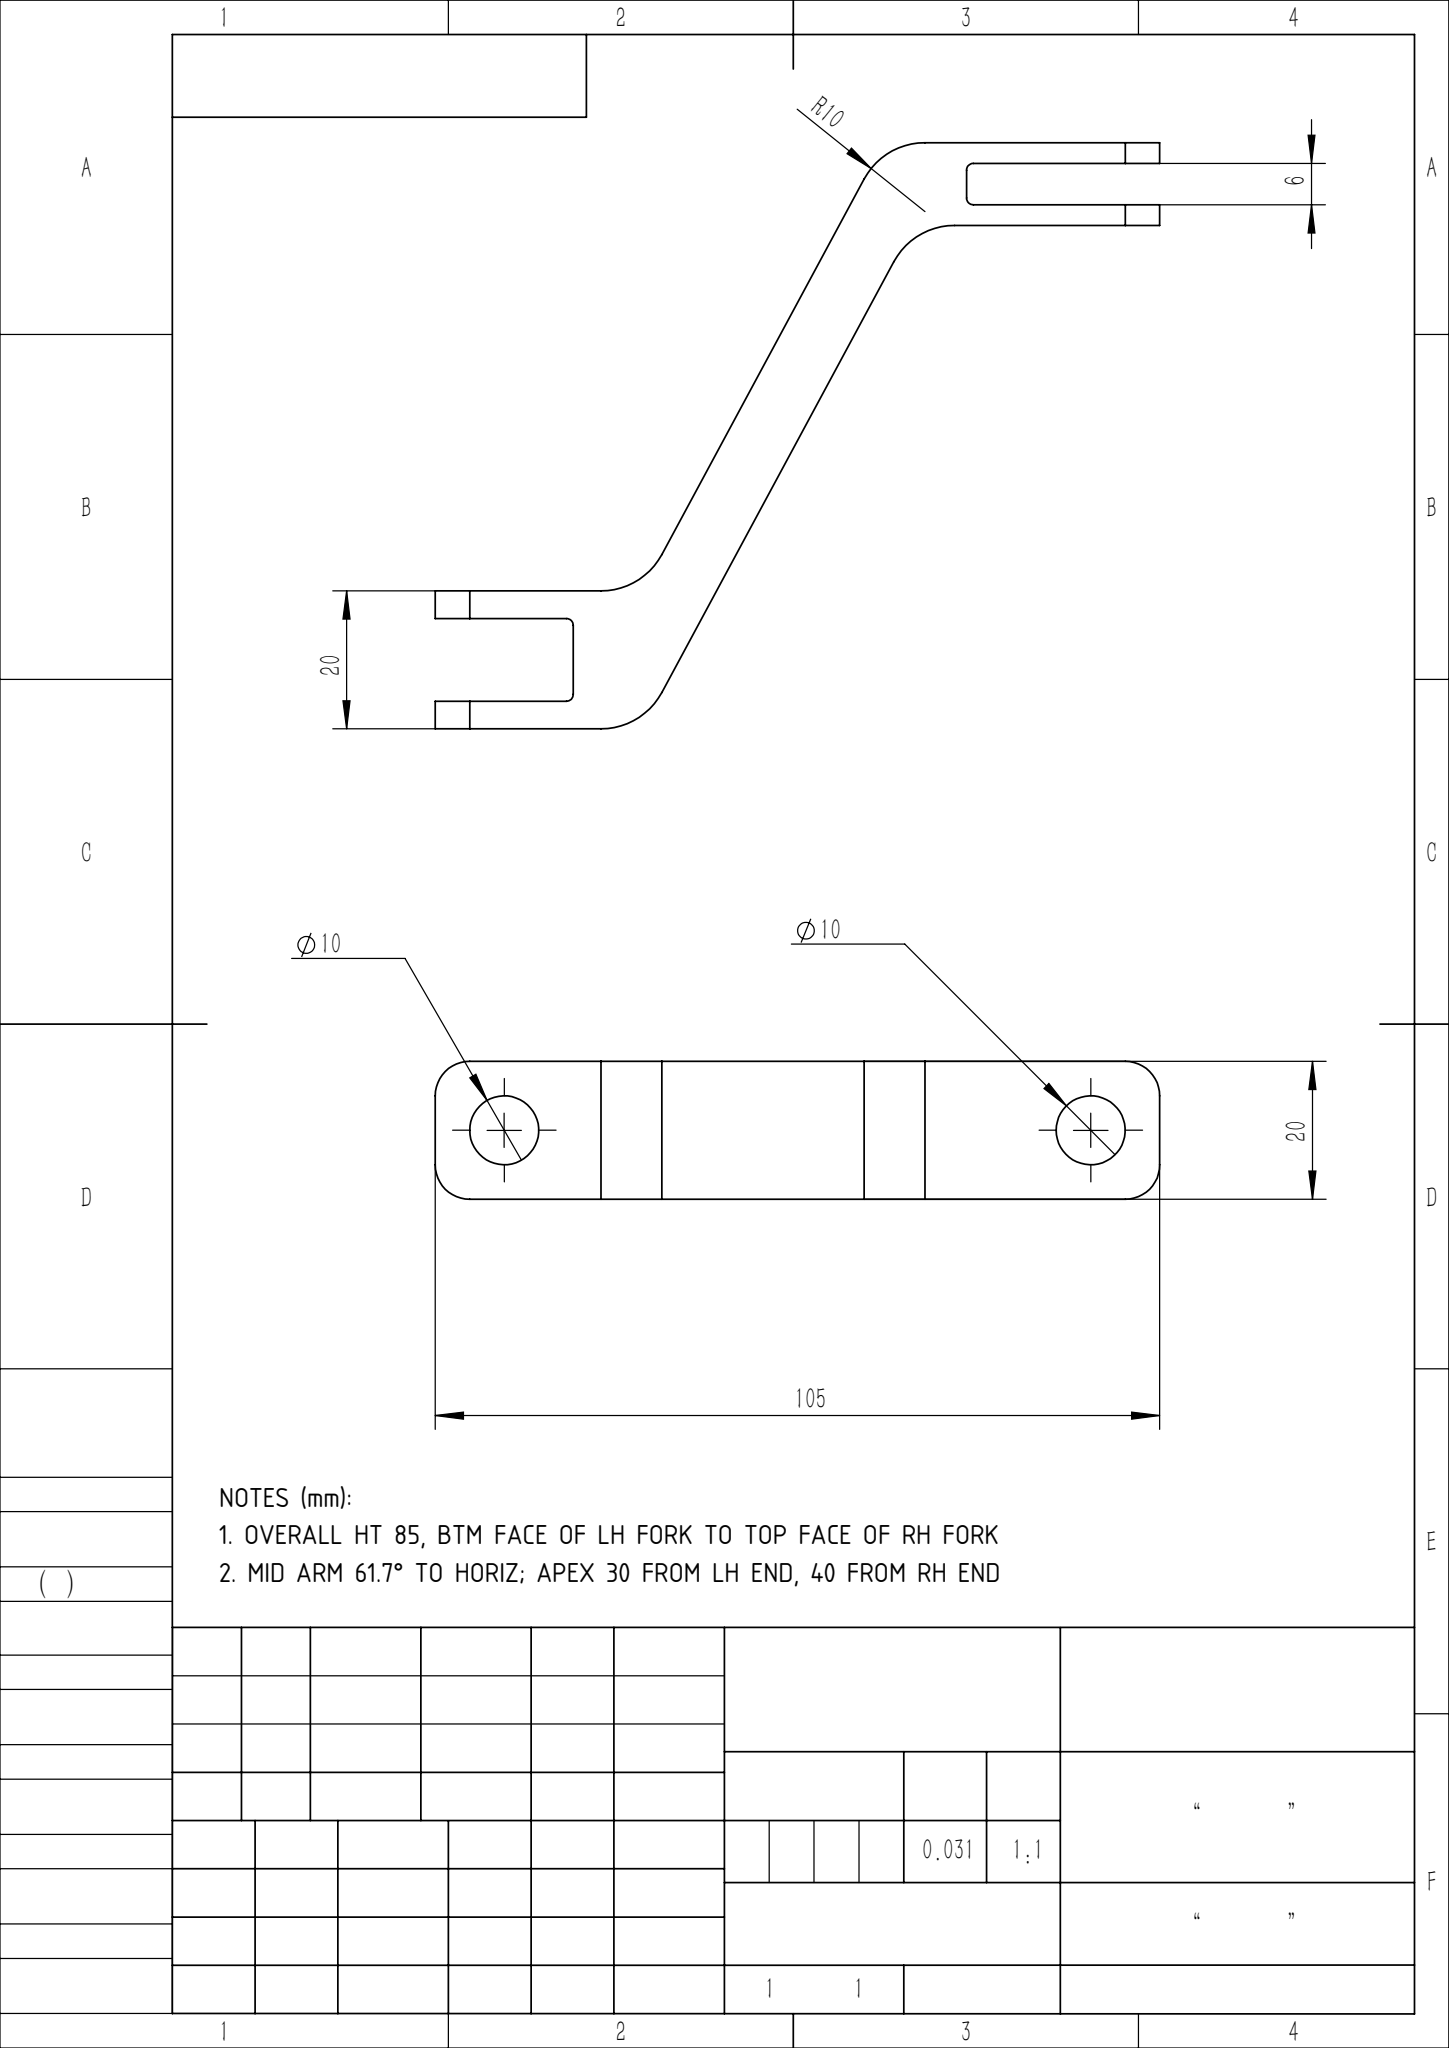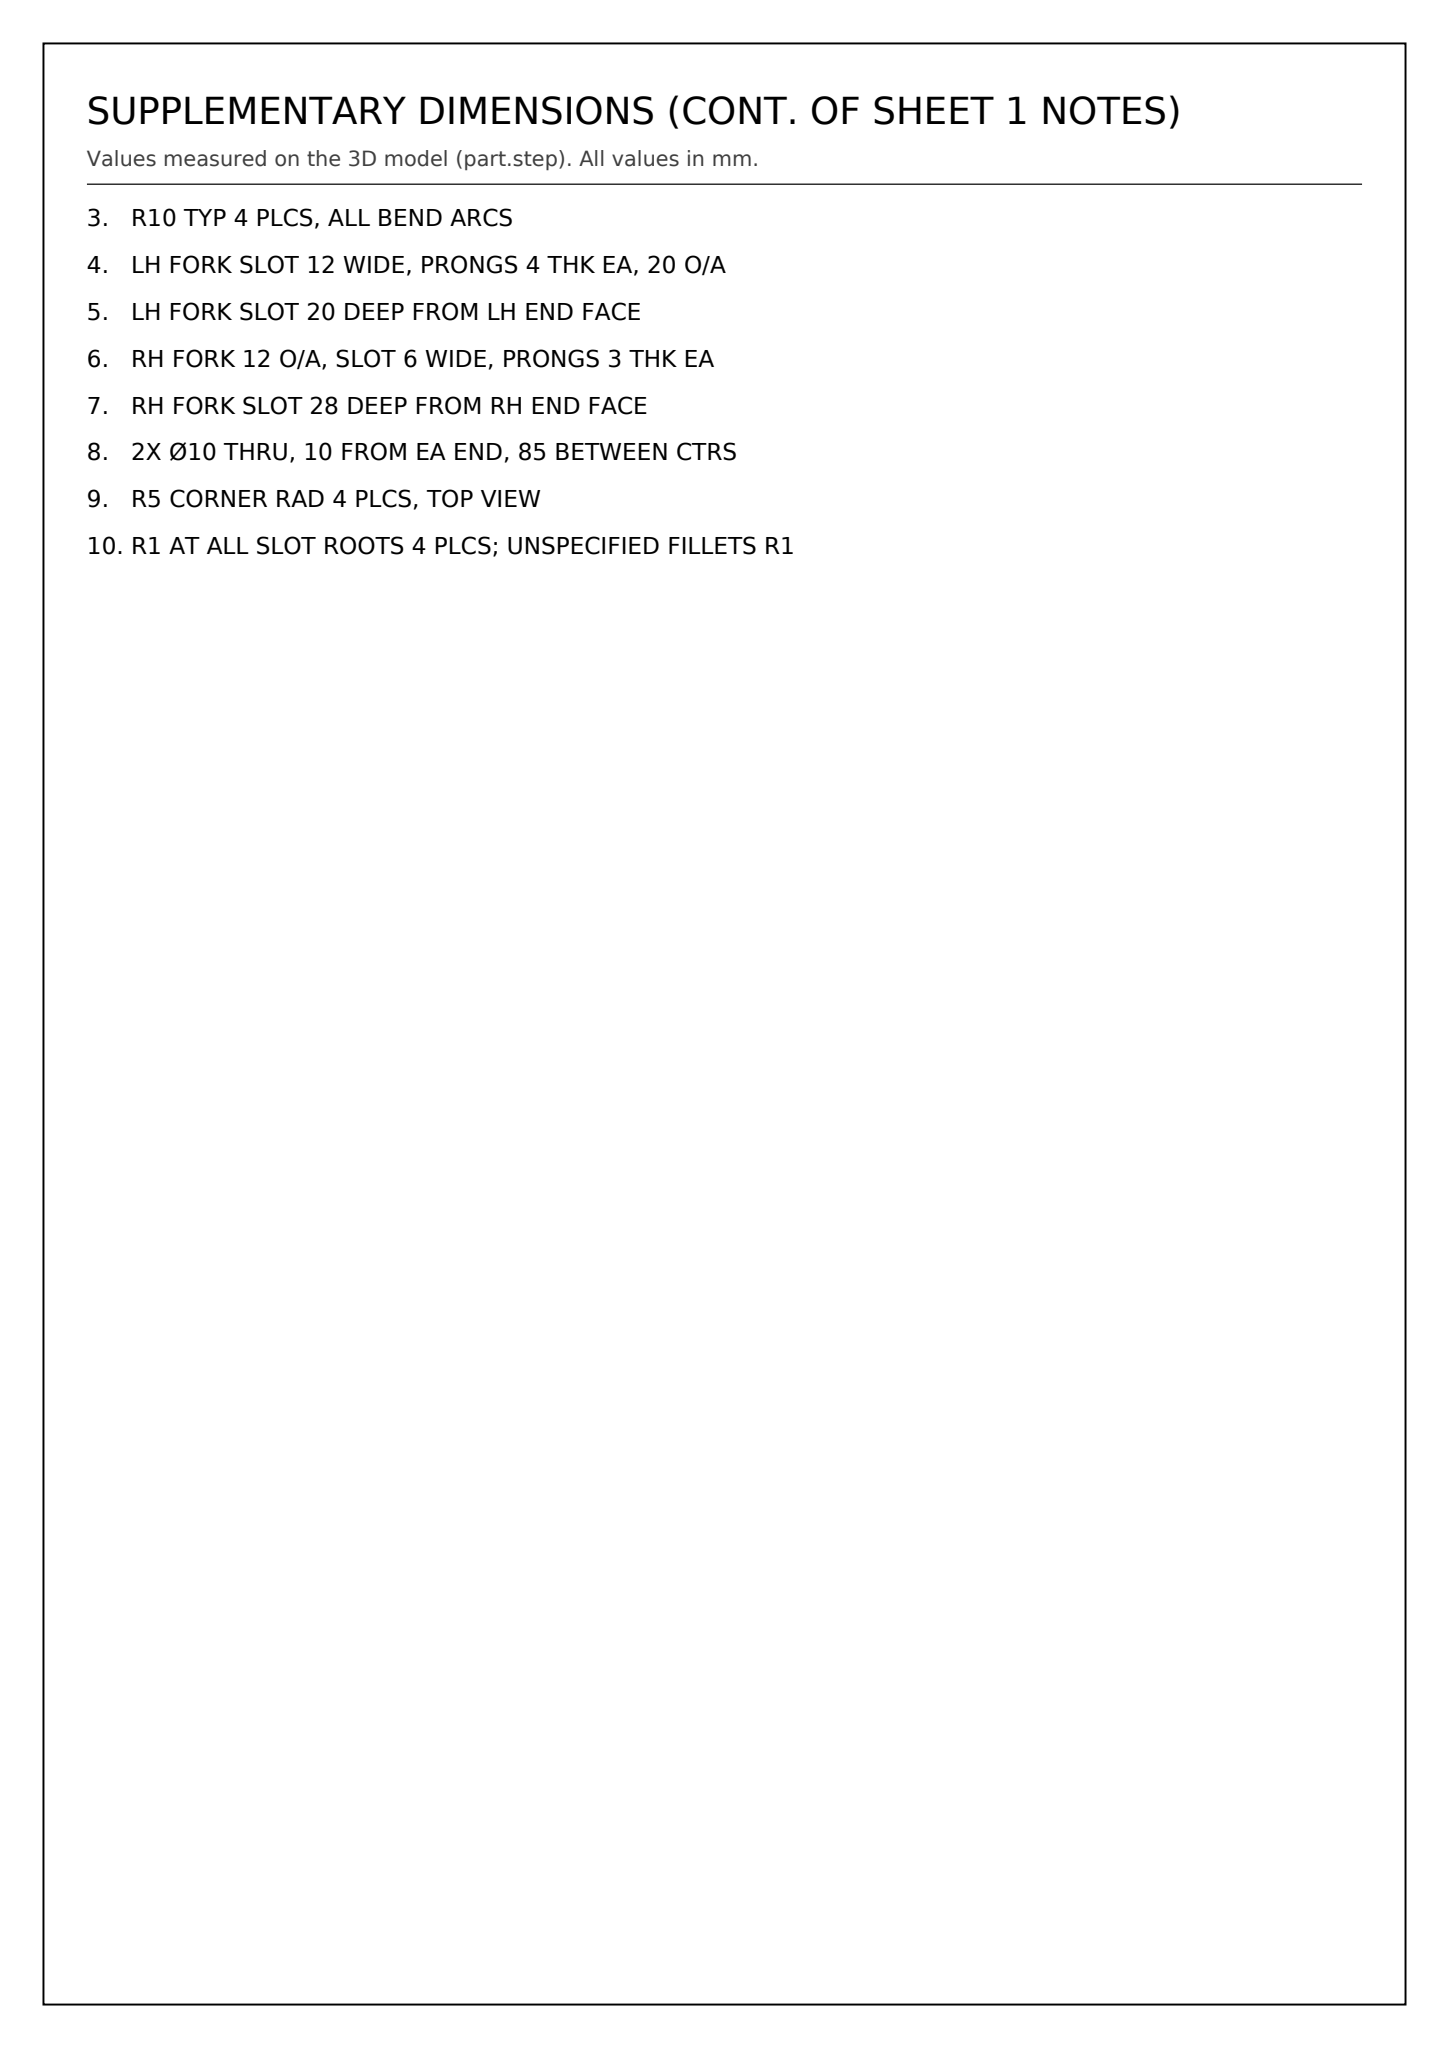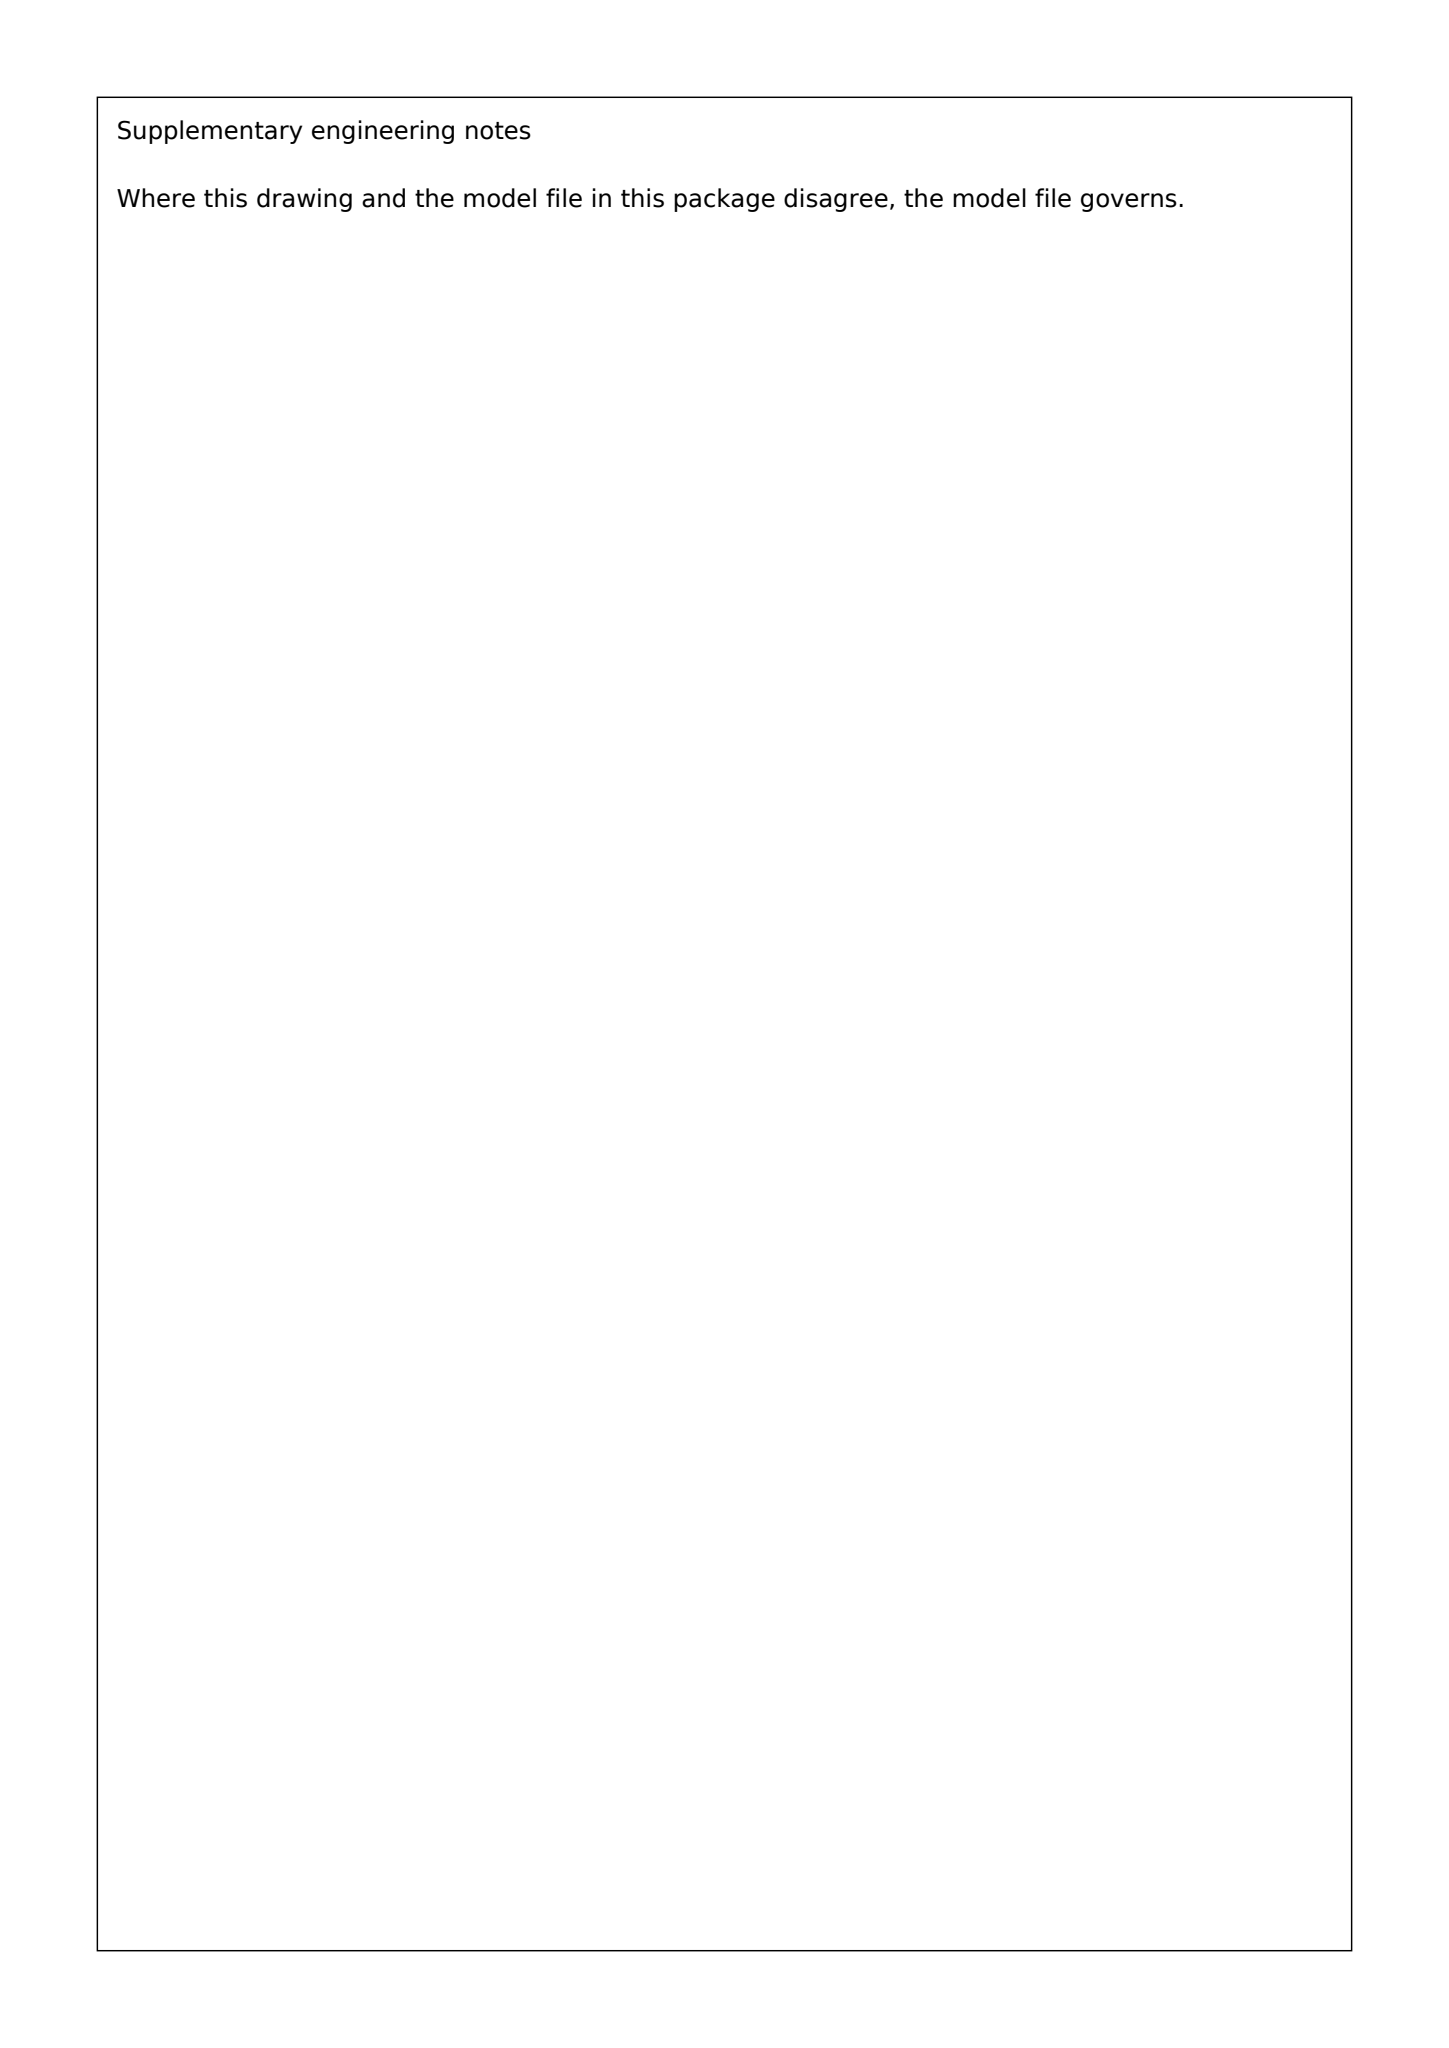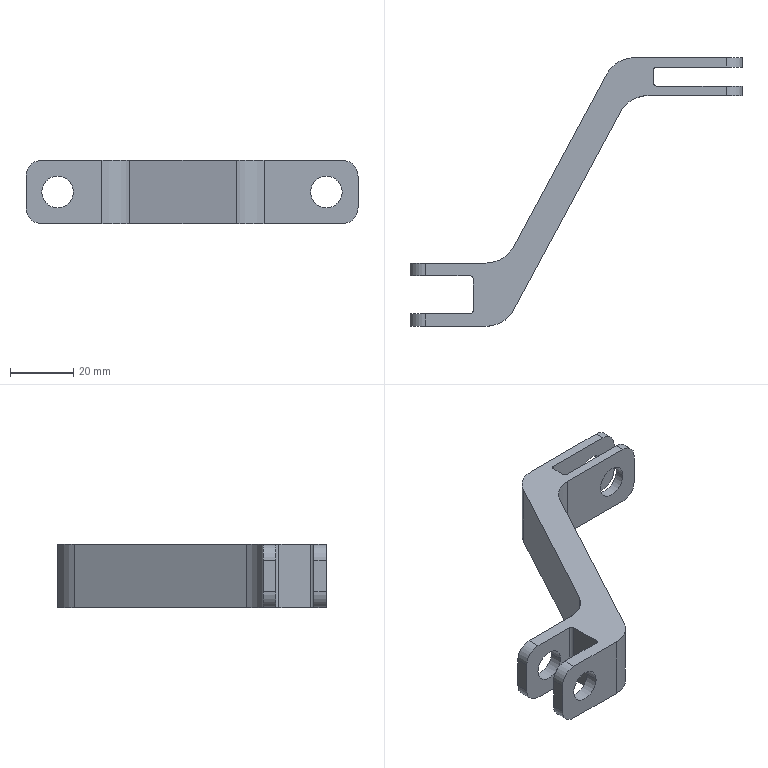Part | SolidWorks | mm | 1 solid | 42 faces | box 105 x 85 x 20 mm | volume 26552 mm3 | cylinder 24 | plane 18 | commonest cylinder face diameters 10 x16 2 x4 20 x4
Drawing notes:
OVERALL HT 85, BTM FACE OF LH FORK TO TOP FACE OF RH FORK | from the solid: bbox_xyz y-extent = 85; planes y=0 and y=85
MID ARM 61.7° TO HORIZ; APEX 30 FROM LH END, 40 FROM RH END | from the solid: R10 bend ctrs (24.03,10)&(75.28,63) and (24.03,30)&(70.97,75) give tan=8/4.31 -> 61.7°; tangent lines meet y=0 at x=30 and y=85 at x=65.0 (=40 from x=105)
R10 TYP 4 PLCS, ALL BEND ARCS | from the solid: four Ø20 z-axis cylinders at (24.03,10),(24.03,30),(70.97,75),(75.28,63)
LH FORK SLOT 12 WIDE, PRONGS 4 THK EA, 20 O/A | from the solid: y-planes 0,4,16,20: slot 4-16 =12, prongs 4 each, overall 20
LH FORK SLOT 20 DEEP FROM LH END FACE | from the solid: x-planes 0 (end) and 20 (slot bottom)
RH FORK 12 O/A, SLOT 6 WIDE, PRONGS 3 THK EA | from the solid: y-planes 73,76,82,85: overall 12, slot 76-82 =6, prongs 3 each
RH FORK SLOT 28 DEEP FROM RH END FACE | from the solid: x-planes 105 (end) and 77 (slot bottom): 105-77=28
2X Ø10 THRU, 10 FROM EA END, 85 BETWEEN CTRS | from the solid: Ø10 y-axis holes at x=10 and x=95, z=10 (C/L of 20 width)
R5 CORNER RAD 4 PLCS, TOP VIEW | from the solid: Ø10 y-axis fillet cyls at (x5,z5),(x5,z15),(x100,z5),(x100,z15)
R1 AT ALL SLOT ROOTS 4 PLCS; UNSPECIFIED FILLETS R1 | from the solid: Ø2 z-axis cyls at (19,5),(19,15),(78,77),(78,81)
build123d program:
from build123d import *

# Parameters (mm, degrees)
SKETCH1_W           = 30
SKETCH1_H           = 20
BOSS_EXTRUDE1_DEPTH = 10
SKETCH2_W           = 20
SKETCH2_H           = 12
SKETCH2_W_2         = 28
SKETCH2_H_2         = 6
CUT_EXTRUDE1_DEPTH  = 39
SKETCH3_R           = 5
CUT_EXTRUDE2_DEPTH  = 39
SKETCH4_R           = 5
CUT_EXTRUDE3_DEPTH  = 39
FILLET1_R           = 1
FILLET2_R           = 5
FILLET3_R           = 10


with BuildPart() as part:
    # Sketch1 → Boss-Extrude1 (new, symmetric)
    with BuildSketch(Plane.XY):
        Polygon((54.308, 63), (15, -10), (15, 10), (50, 75), (90, 75), (90, 63), align=None)
        Rectangle(SKETCH1_W, SKETCH1_H)
    extrude(amount=BOSS_EXTRUDE1_DEPTH, both=True)

    # Sketch2 → Cut-Extrude1 (cut)
    with BuildSketch(Plane.XY.offset(10)):
        with Locations((-5, 0)):
            Rectangle(SKETCH2_W, SKETCH2_H)
        with Locations((76, 69)):
            Rectangle(SKETCH2_W_2, SKETCH2_H_2)
    extrude(amount=-CUT_EXTRUDE1_DEPTH, mode=Mode.SUBTRACT)

    # Sketch3 → Cut-Extrude2 (cut)
    with BuildSketch(Plane(origin=(0, 10, 0), x_dir=(1, 0, 0), z_dir=(0, 1, 0))):
        with Locations((-5, 0)):
            Circle(SKETCH3_R)
    extrude(amount=-CUT_EXTRUDE2_DEPTH, mode=Mode.SUBTRACT)

    # Sketch4 → Cut-Extrude3 (cut)
    with BuildSketch(Plane(origin=(0, 75, 0), x_dir=(1, 0, 0), z_dir=(0, 1, 0))):
        with Locations(Location((80, 0, 0), (0, 0, 180))):
            Circle(SKETCH4_R)
    extrude(amount=-CUT_EXTRUDE3_DEPTH, mode=Mode.SUBTRACT)

    # Fillet1
    fillet1_edges = [part.edges().sort_by_distance(p)[0] for p in [
        (5, 6, 0),
        (5, -6, 0),
        (62, 66, 0),
        (62, 72, 0),
    ]]
    fillet(fillet1_edges, radius=FILLET1_R)

    # Fillet2
    fillet2_edges = [part.edges().sort_by_distance(p)[0] for p in [
        (-15, -8, -10),
        (90, 73.5, -10),
        (90, 73.5, 10),
        (-15, 8, -10),
        (90, 64.5, -10),
        (90, 64.5, 10),
        (-15, 8, 10),
        (-15, -8, 10),
    ]]
    fillet(fillet2_edges, radius=FILLET2_R)

    # Fillet3
    fillet3_edges = [part.edges().sort_by_distance(p)[0] for p in [
        (15, -10, 0),
        (15, 10, 0),
        (50, 75, 0),
        (54.308, 63, 0),
    ]]
    fillet(fillet3_edges, radius=FILLET3_R)


solid = part.part